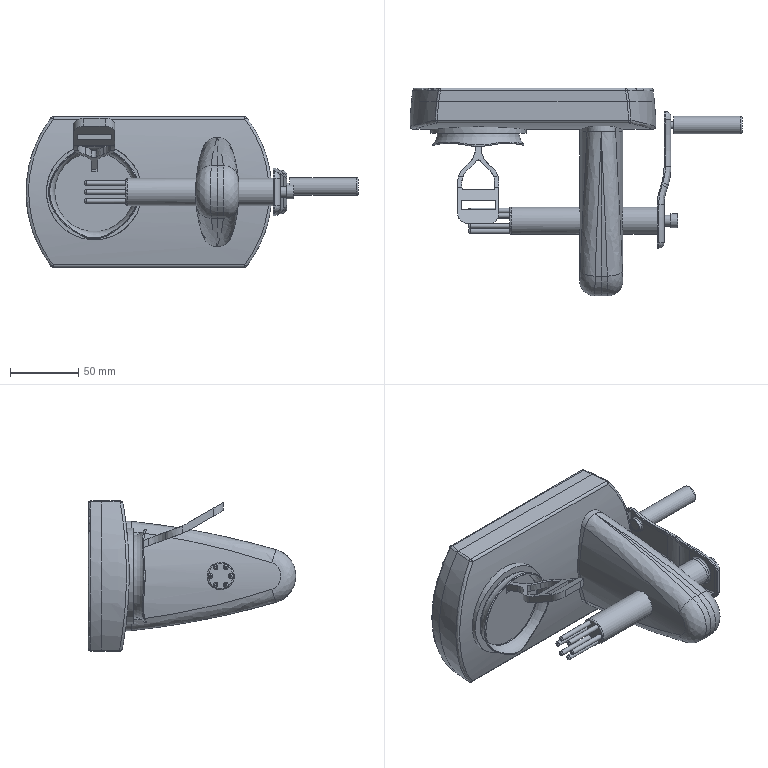Assembly | NX | mm | 9 component files | 9 solids | 371 faces | box 242.99 x 152 x 110 mm | volume 215533 mm3 | cylinder 124 | plane 122 | spline 72 | torus 27 | sphere 12 | cone 10 | other 4 | commonest cylinder face diameters 4 x13 200 x8 8 x7 10 x7 100 x6 3.5 x6 20 x5 80 x4
Bill of materials:
unnamed part 1 | 1 |  | Thin flat plate-like part. One end is a wide, rounded-rectangle loop and the other end is a narrow straight tail. The loop has a straight rectangular slot through it and a larger open window with a contoured, V-shaped edge where it joins the tail. In side view the part bends slightly along its length.
unnamed part 2 | 1 |  | Solid cylindrical pin with a small chamfer or round on one end. The other end has a short, smaller-diameter stub, and a narrower neck or groove separates the stub from the main body.
unnamed part 3 | 1 |  | Thin strap or bar with rounded edges and an S-shaped joggle (offset bend) in the middle. One end has a larger round through-hole and the other end has a smaller one. The width narrows slightly around the middle.
unnamed part 4 | 1 |  | Thin flat plate with two straight parallel edges and two convex arc ends, plus chamfered corners. One face has a raised rim around its edge. At the center there is a small round boss with a hole, surrounded by four small radial ribs or tabs in a cross pattern.
unnamed part 5 | 1 |  | Solid, tapered teardrop or tongue-shaped slab. One end is rounded and the other is wide and cut off. It has one circular through-hole near the rounded end. One face is domed or curved and the other appears flat.
unnamed part 6 | 1 |  | Thick flat plate with two straight parallel sides and two convex arc ends. One face has a large shallow circular boss or recess with concentric rings, and next to it is an elongated oval through-slot with a raised lip. Short bosses stick out from the underside below both features.
unnamed part 7 | 1 |  | Thin-walled, open shell with a tapered teardrop outline and an outward-curved (convex) back. It has a cylindrical boss with a through-hole near the rounded end, and the open, wide end is cut off. Its outline matches the solid tapered part (unnamed part 5), but it is hollow.
unnamed part 8 | 1 |  | Long, stepped cylindrical body made of a revolved shape. One end has several thin parallel pins (about five) sticking out lengthwise. Partway along the body is a thin collar or flange. The other end has a hex-like section followed by a smaller stepped round stub.
unnamed part 9 | 1 |  | Shallow, thin-walled ring or bezel-like shell. It has a flat, roughly circular plate on one face, a rounded-square outer lip, and a curved, flaring side wall. There is a small rectangular opening near one edge of the flat plate, and the lip edge rises and falls in a wave in the side view.
Mates:
1. touch align | front_casing 1 face | upper_casing 1 face
2. touch align | rear_casing 1 face | upper_casing 1 face
3. touch align | rear_casing 1 face | front_casing 1 face
4. touch align | rear_casing 1 face | front_casing 1 face
5. touch align | lower_casing 1 face | upper_casing 1 face
6. touch align | lower_casing 1 edge | upper_casing 1 edge
7. touch align | fruit_tray 1 face | upper_casing 1 face
8. touch align | fruit_tray 1 edge | upper_casing 1 face
9. touch align | blade 1 face | upper_casing 1 face
10. touch align | blade 1 face | fruit_tray 1 face
11. distance | blade 1 face | fruit_tray 1 edge
12. touch align | shaft_01 1 face | rear_casing 1 face
13. touch align | shaft_01 1 face | rear_casing 1 face
14. touch align | handle 1 face | shaft_01 1 face
15. touch align | handle 1 edge | shaft_01 1 face
16. touch align | shaft_02 1 face | handle 1 face
17. touch align | shaft_02 1 face | handle 1 face